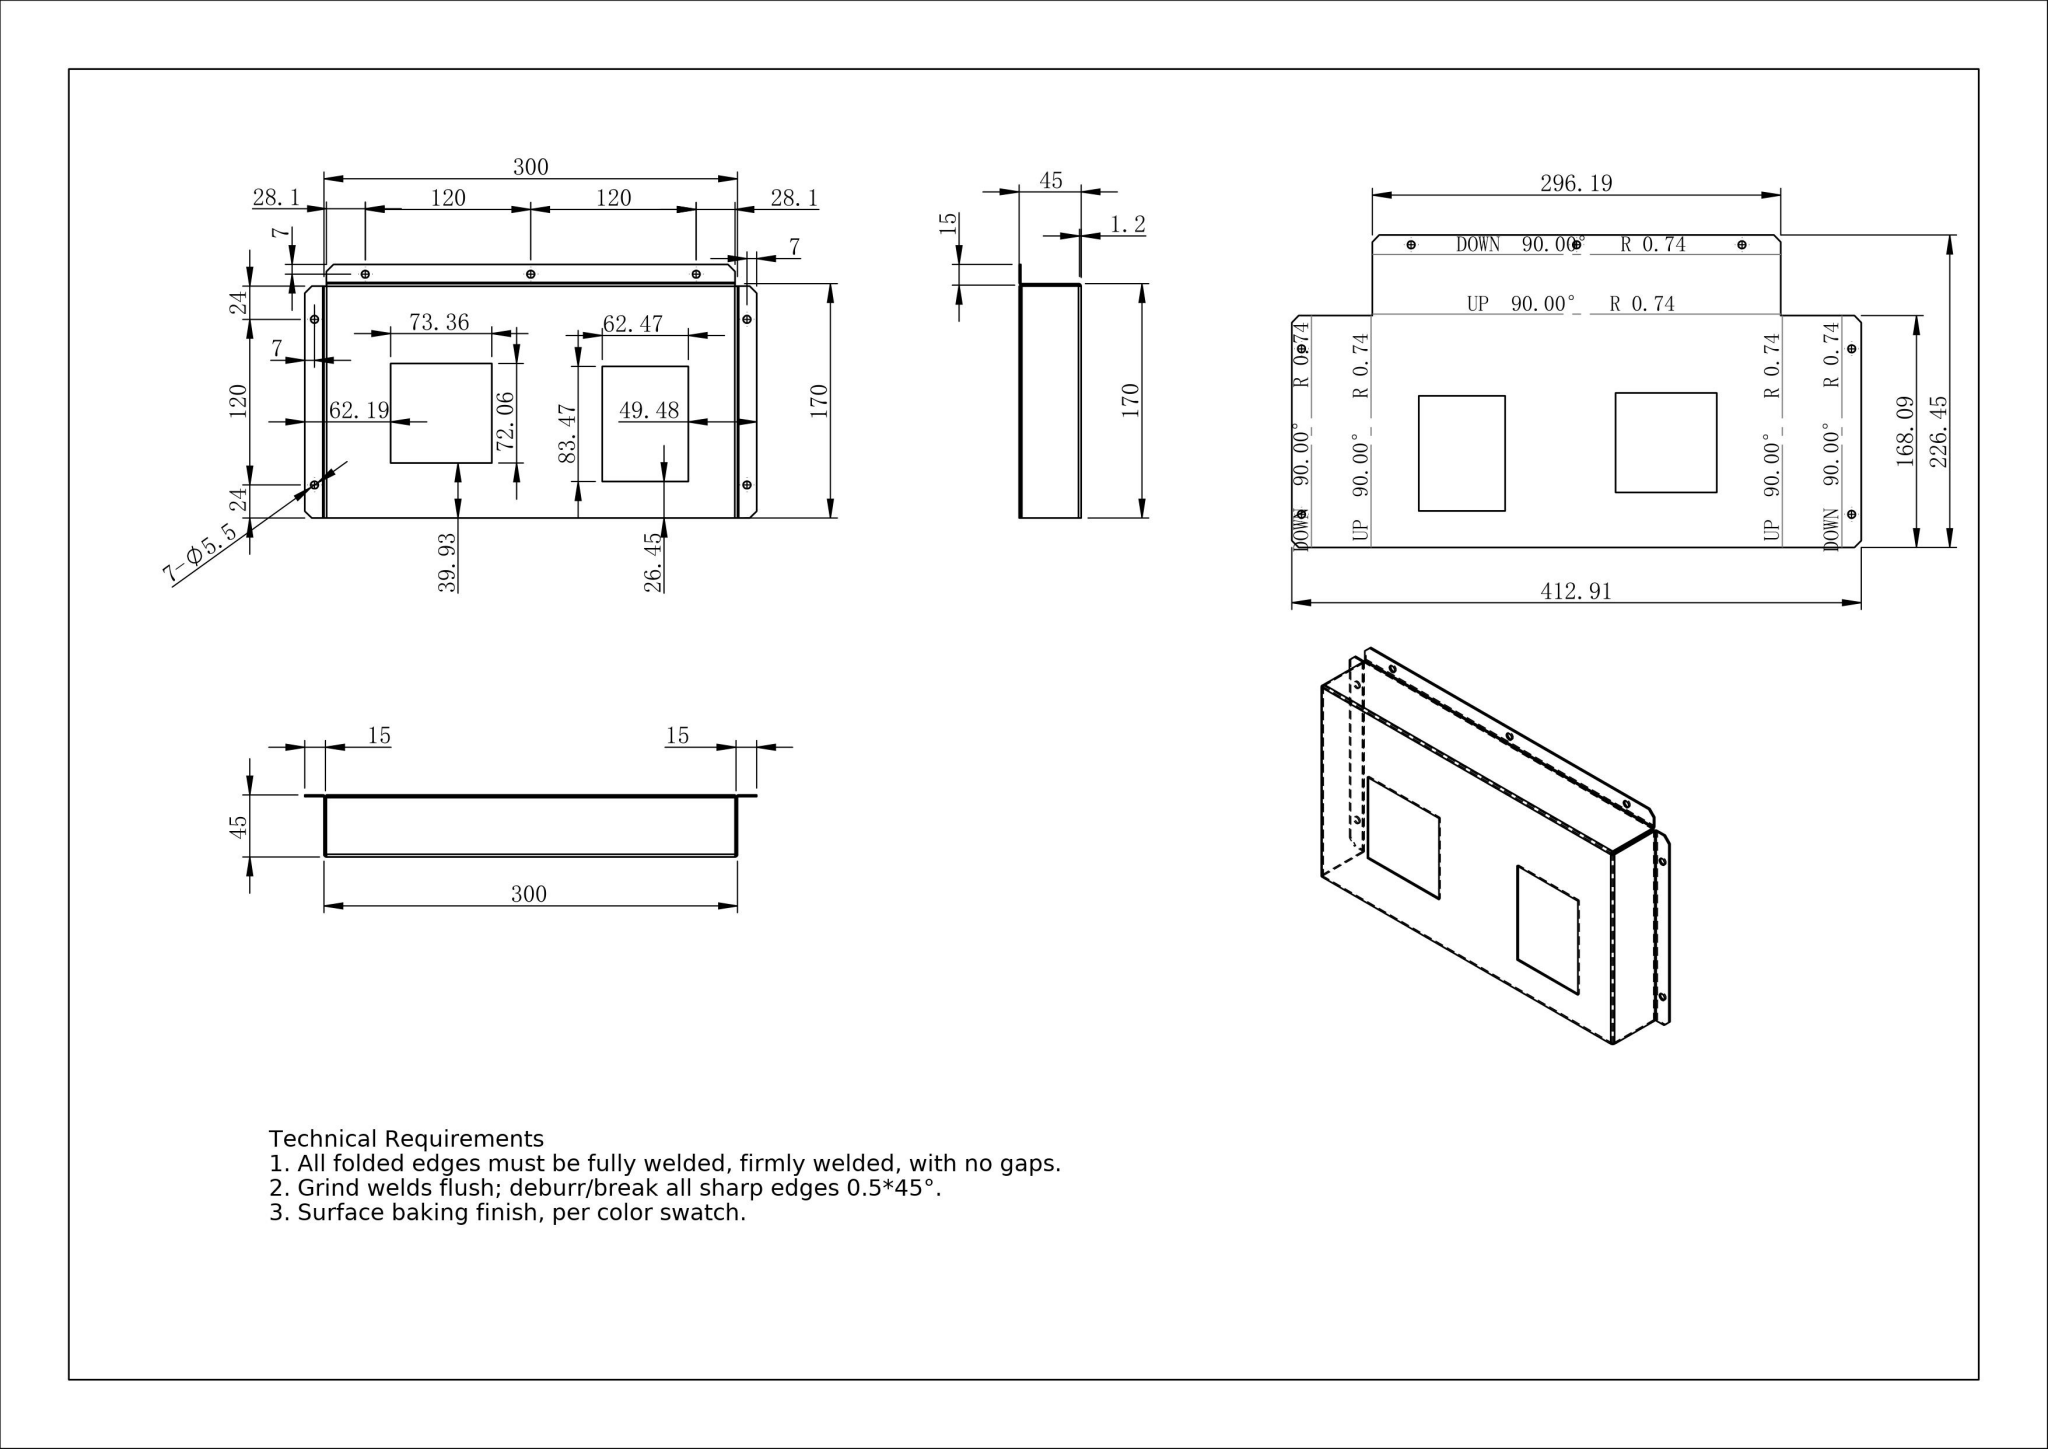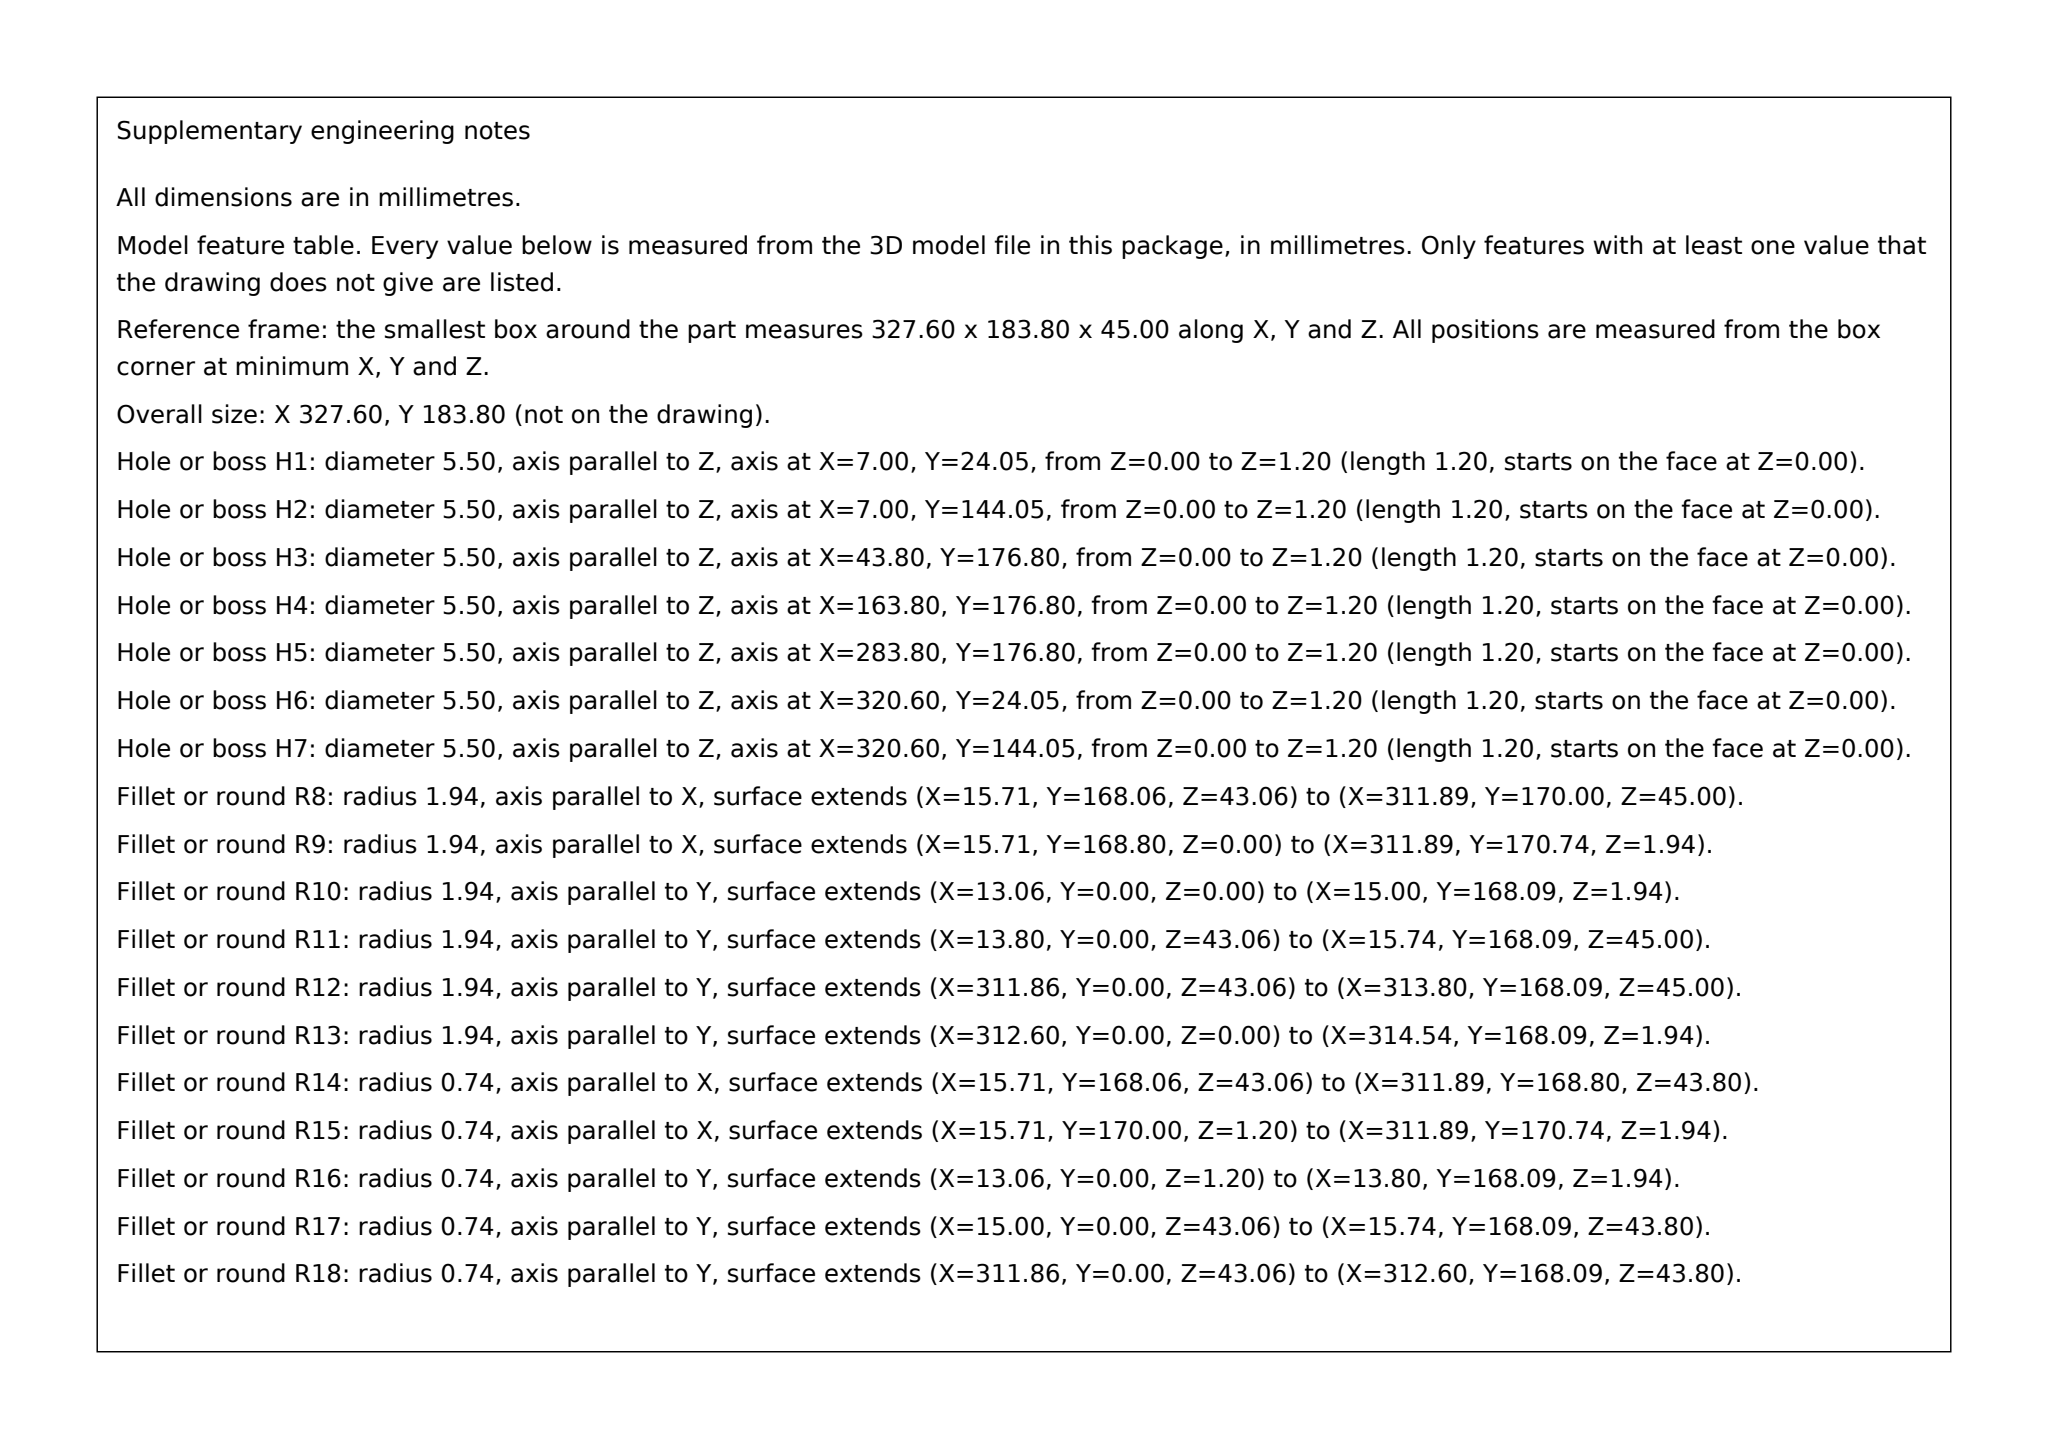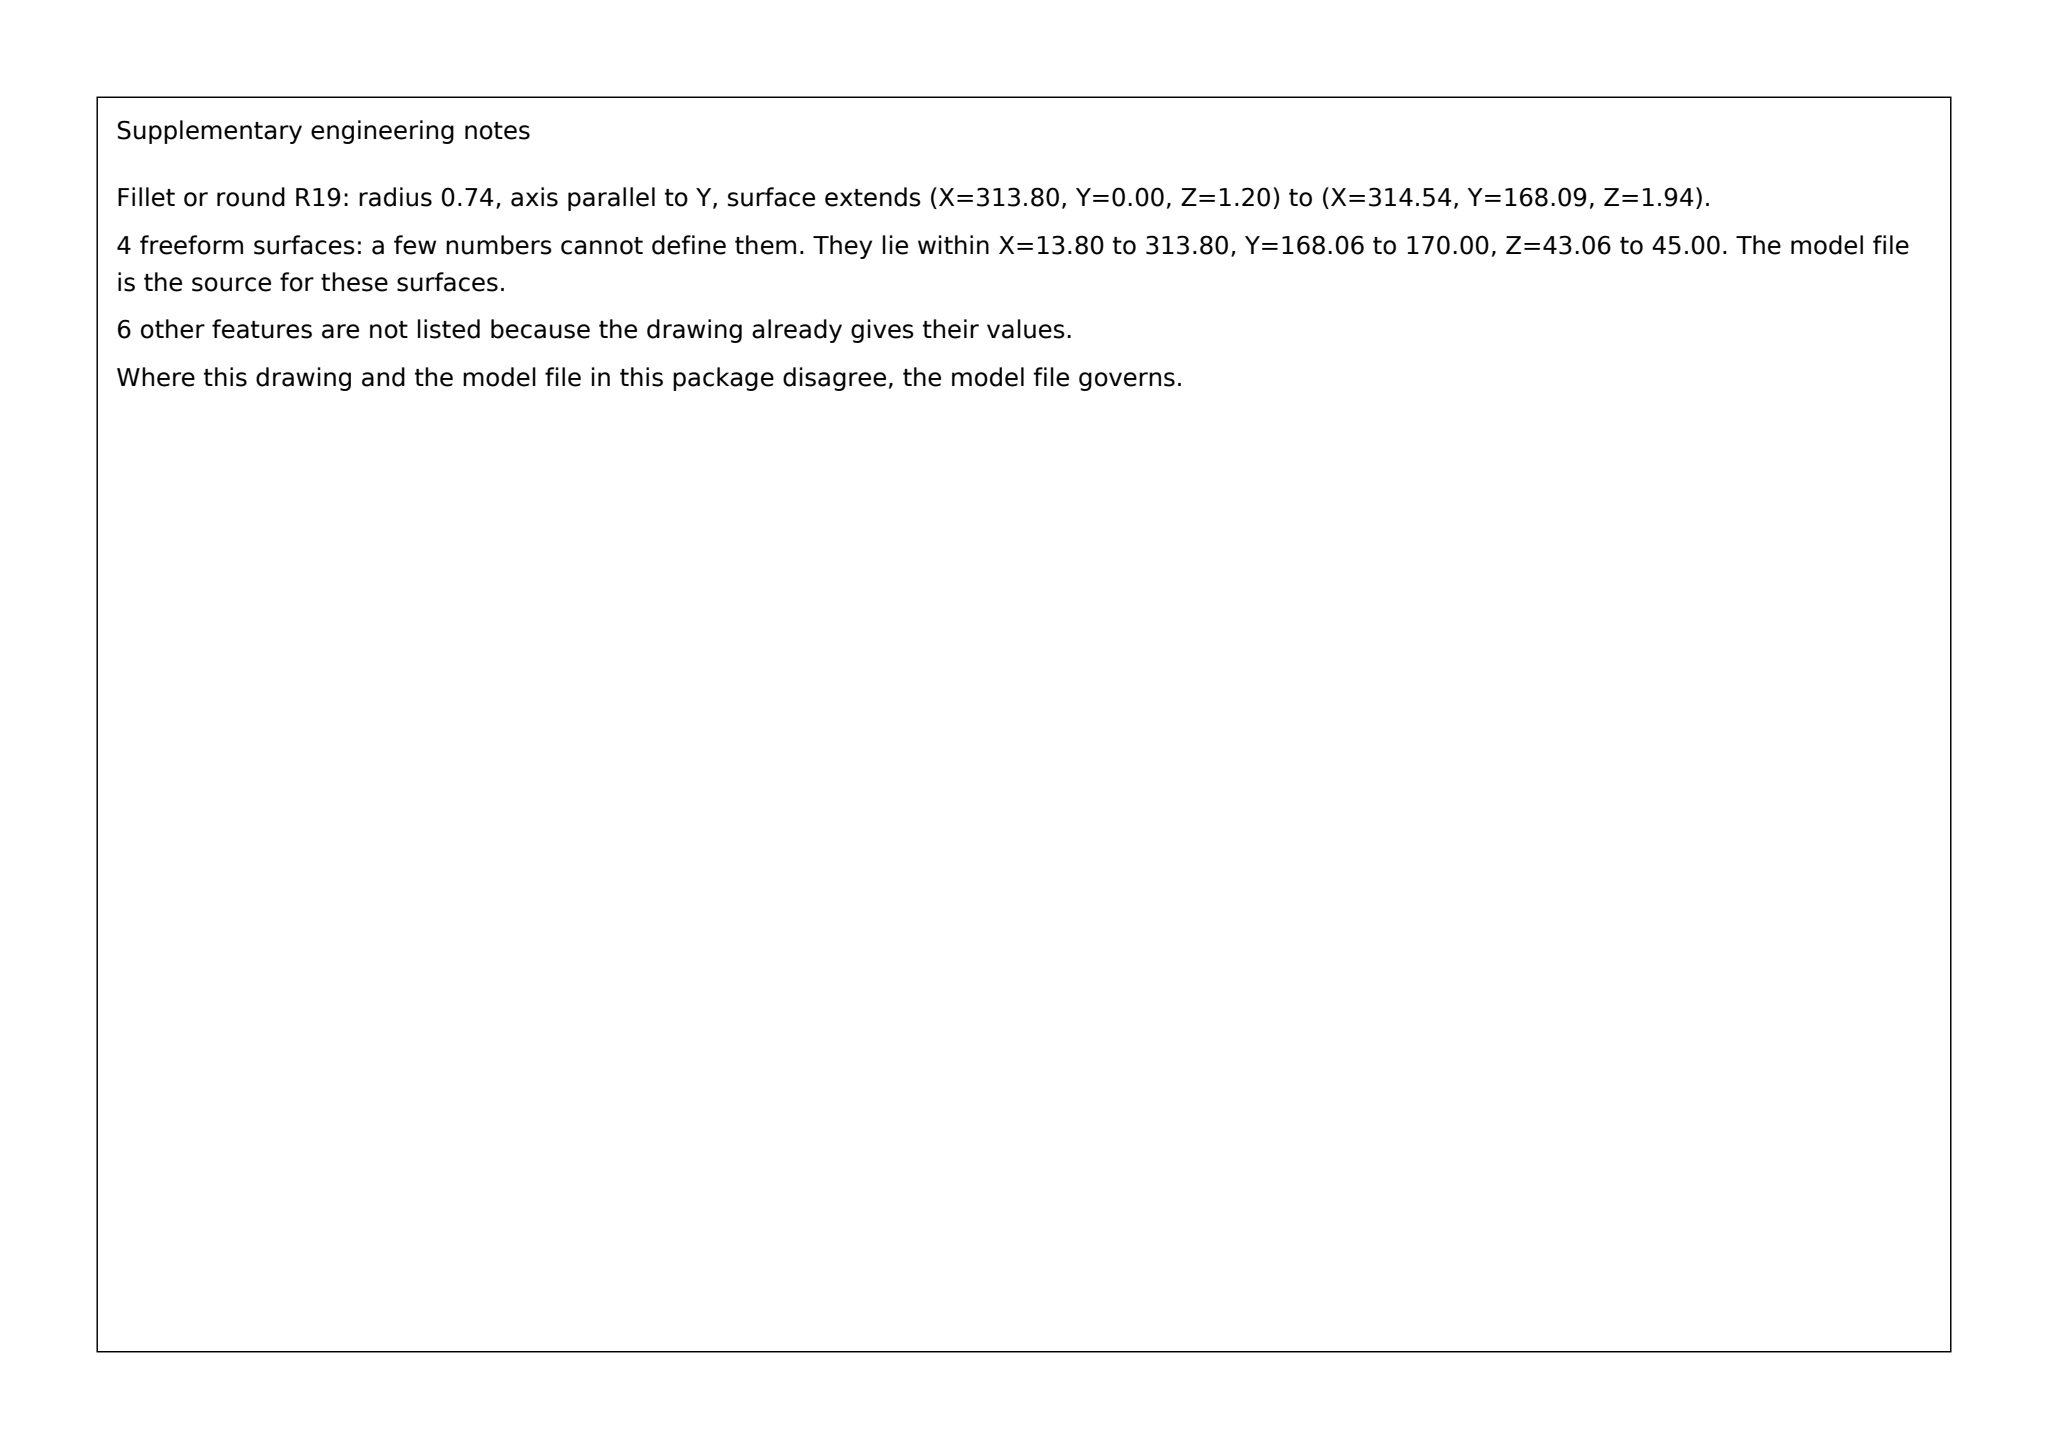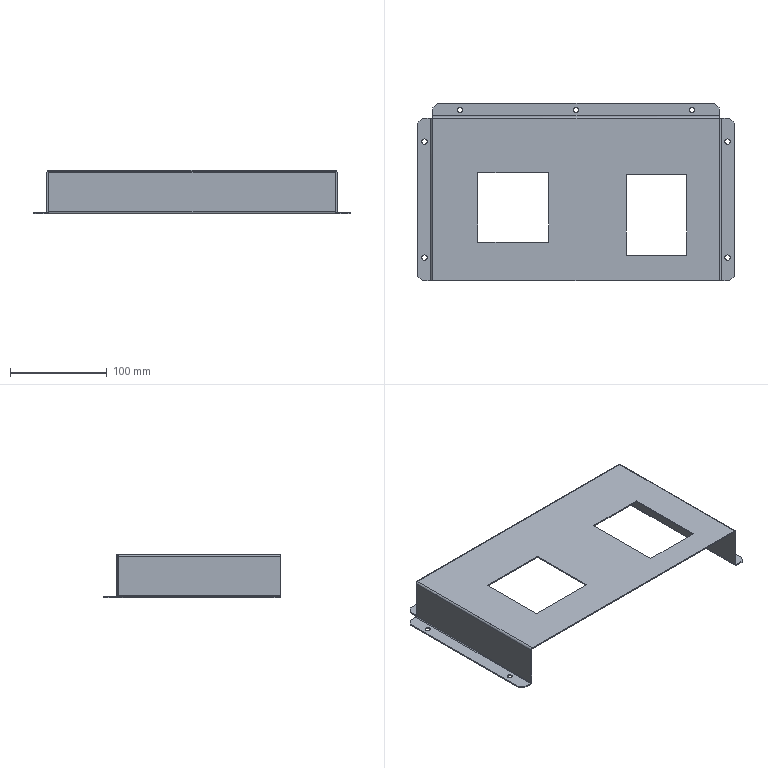Part | SolidWorks | mm | 1 solid | 82 faces | box 327.6 x 183.8 x 45 mm | volume 91139 mm3 | plane 52 | cylinder 26 | spline 4 | commonest cylinder face diameters 5.5 x14 3.873 x6 1.473 x6